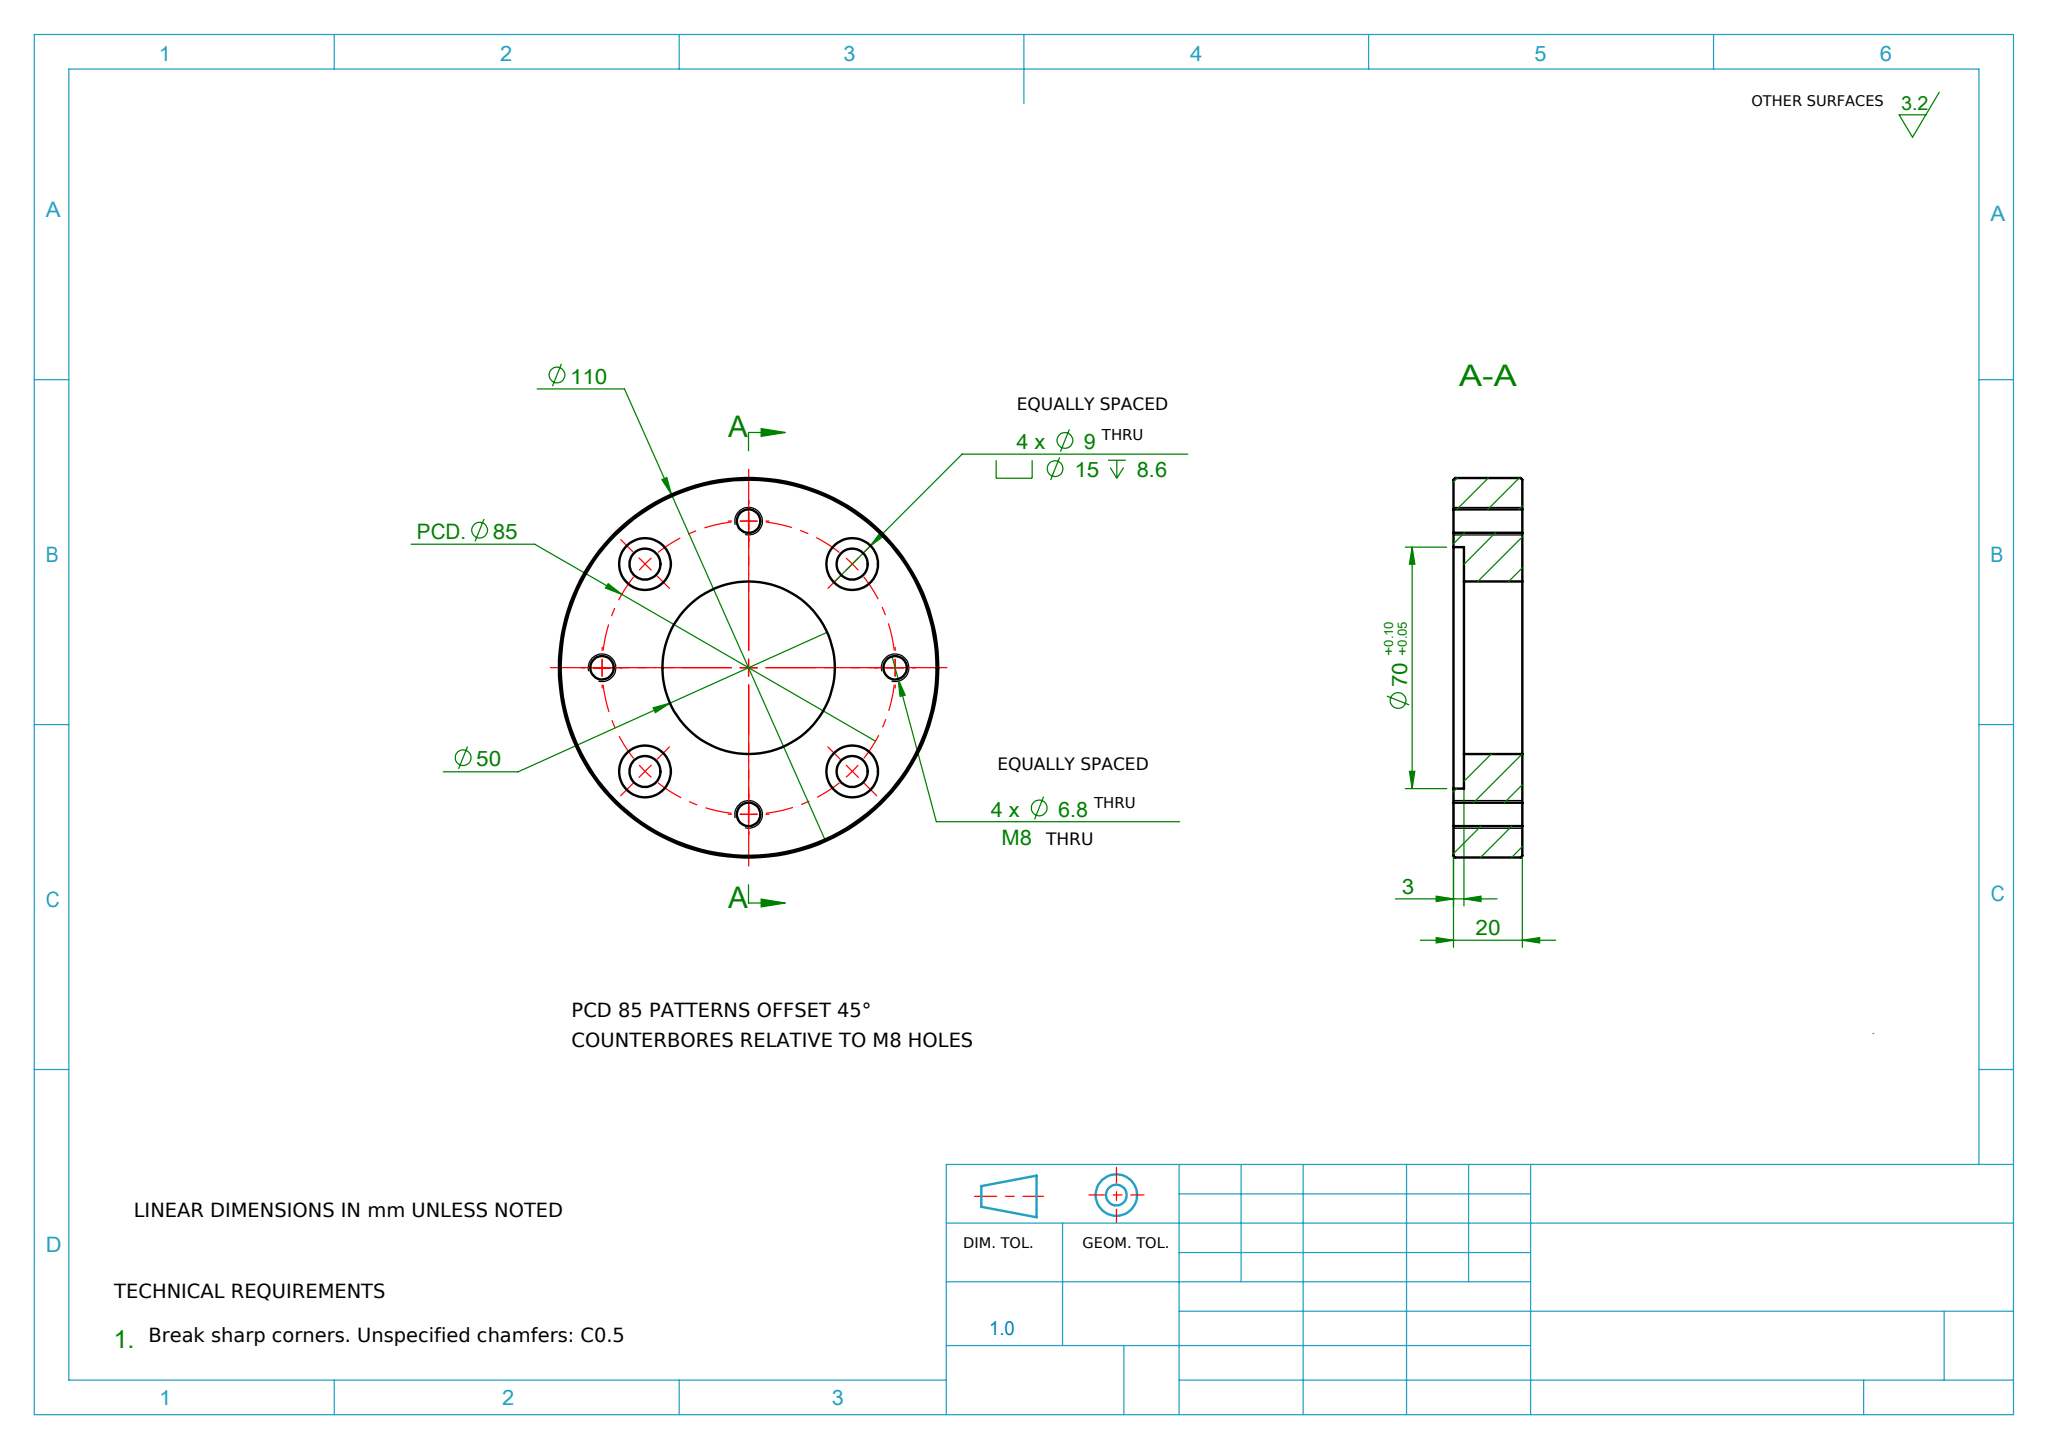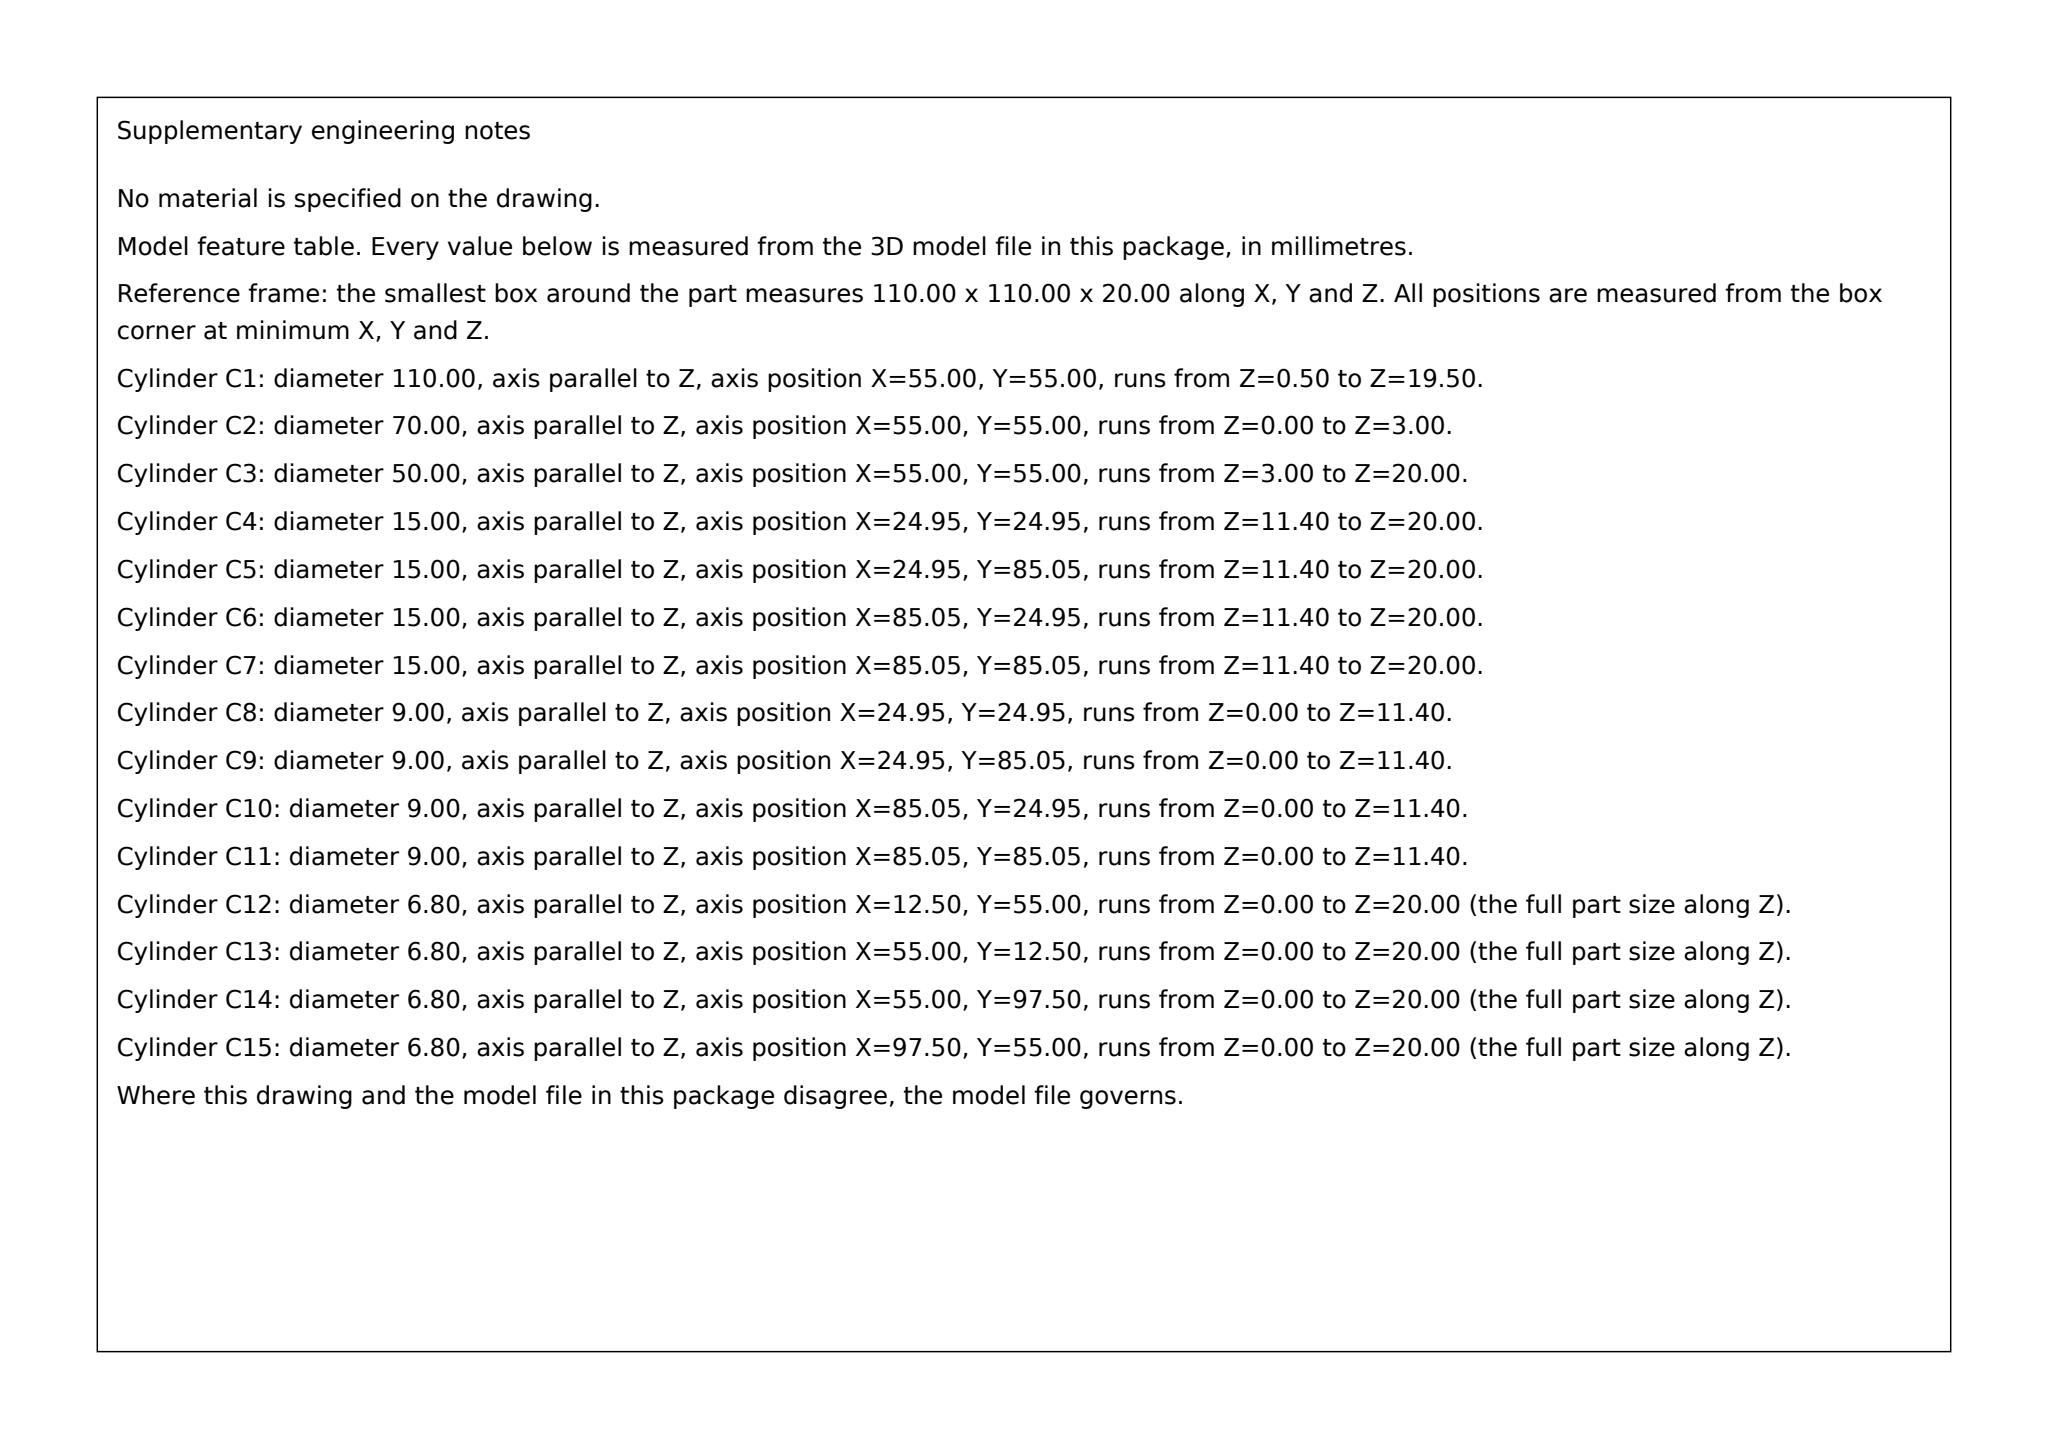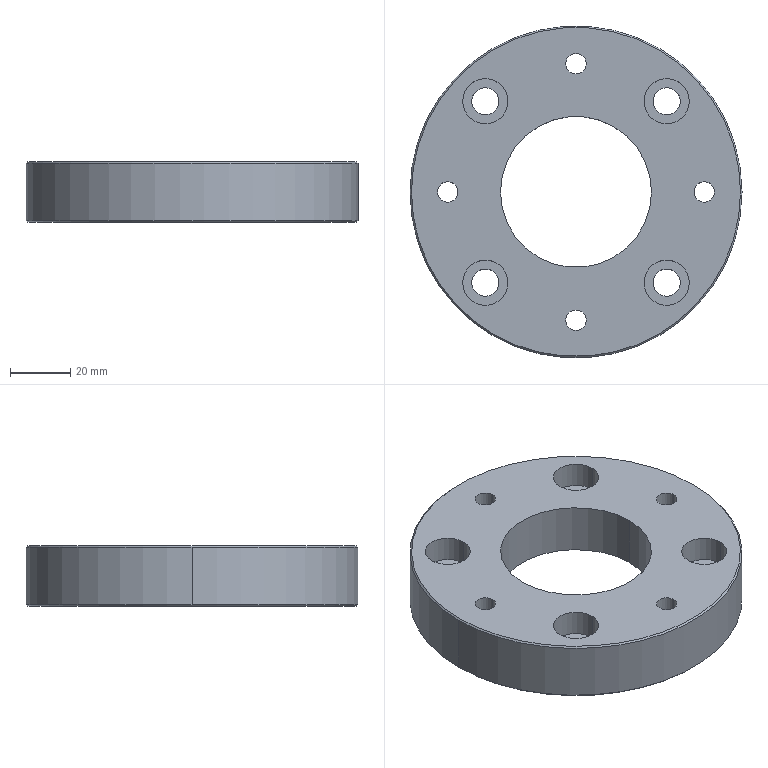Part | SolidWorks | mm | 1 solid | 41 faces | box 110 x 110 x 20 mm | volume 133170 mm3 | cylinder 30 | plane 7 | cone 4 | commonest cylinder face diameters 6.8 x8 15 x8 9 x8 50 x2 70 x2 110 x2
build123d program:
from build123d import *

# Parameters (mm, degrees)
SKETCH1_R                                       = 55
BOSS_EXTRUDE1_DEPTH                             = 20
SKETCH2_R                                       = 35
CUT_EXTRUDE1_DEPTH                              = 3
SKETCH3_R                                       = 25
CUT_EXTRUDE2_DEPTH                              = 80.618
M8_HEX_SOCKET_HEAD_CAP_SCREW_CBORE8_D           = 9
M8_HEX_SOCKET_HEAD_CAP_SCREW_CBORE8_CBORE_D     = 15
M8_HEX_SOCKET_HEAD_CAP_SCREW_CBORE8_CBORE_DEPTH = 8.6
M8_TAPPED_HOLE1_D                               = 6.8
CHAMFER1_SIZE                                   = 0.5


with BuildPart() as part:
    # Sketch1 → Boss-Extrude1 (new body)
    with BuildSketch(Plane.XY):
        Circle(SKETCH1_R)
    extrude(amount=BOSS_EXTRUDE1_DEPTH)

    # Sketch2 → Cut-Extrude1 (cut)
    with BuildSketch(Plane(origin=(0, 0, 0), x_dir=(-1, 0, 0), z_dir=(0, 0, -1))):
        Circle(SKETCH2_R)
    extrude(amount=-CUT_EXTRUDE1_DEPTH, mode=Mode.SUBTRACT)

    # Sketch3 → Cut-Extrude2 (cut, through all)
    with BuildSketch(Plane(origin=(0, 0, 3), x_dir=(-1, 0, 0), z_dir=(0, 0, -1))):
        Circle(SKETCH3_R)
    extrude(amount=-CUT_EXTRUDE2_DEPTH, mode=Mode.SUBTRACT)

    # M8 Hex Socket Head Cap Screw CBORE8 (through all)
    with Locations(Plane.XY.offset(20)):
        with Locations((-30.052, -30.052), (-30.052, 30.052), (30.052, -30.052), (30.052, 30.052)):
            CounterBoreHole(M8_HEX_SOCKET_HEAD_CAP_SCREW_CBORE8_D / 2, M8_HEX_SOCKET_HEAD_CAP_SCREW_CBORE8_CBORE_D / 2, M8_HEX_SOCKET_HEAD_CAP_SCREW_CBORE8_CBORE_DEPTH)

    # M8 Tapped Hole1 (through all)
    with Locations(Plane.XY.offset(20)):
        with Locations((-42.5, 0), (0, -42.5), (42.5, 0), (0, 42.5)):
            Hole(M8_TAPPED_HOLE1_D / 2)

    # Chamfer1
    chamfer1_edges = [part.edges().sort_by_distance(p)[0] for p in [
        (-55, 0, 0),
        (-55, 0, 20),
    ]]
    chamfer(chamfer1_edges, length=CHAMFER1_SIZE)


solid = part.part